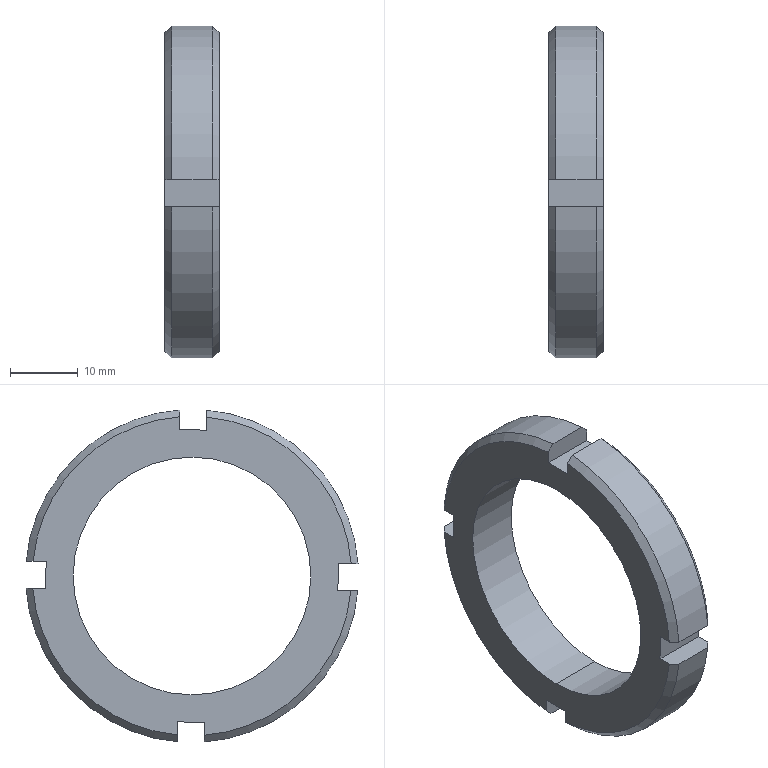Component | SolidWorks | 2-10-10WorkpieceAxisAssembly-1_2-10-5LockNut-1 | 1 solid | 28 faces | box 8 x 48.87 x 48.87 mm | volume 6873 mm3 | plane 14 | cone 8 | cylinder 6 | commonest cylinder face diameters 49 x4 35 x2
STEP:
#1=CARTESIAN_POINT('',(-19.953,-0.1704,0.689));
#2=VERTEX_POINT('',#1);
#3=CARTESIAN_POINT('',(-19.953,-0.1588,-0.689));
#4=VERTEX_POINT('',#3);
#5=CARTESIAN_POINT('',(-19.953,-0.1646,-0.));
#6=DIRECTION('',(1.,-0.,0.));
#7=DIRECTION('',(0.,0.008395,-1.));
#8=AXIS2_PLACEMENT_3D('',#5,#6,#7);
#9=CIRCLE('',#8,0.689);
#10=EDGE_CURVE('',#2,#4,#9,.T.);
#11=ORIENTED_EDGE('',*,*,#10,.F.);
#12=CARTESIAN_POINT('',(-19.638,-0.1704,0.689));
#13=VERTEX_POINT('',#12);
#14=CARTESIAN_POINT('',(-19.638,-0.1704,0.689));
#15=DIRECTION('',(1.,-0.,0.));
#16=VECTOR('',#15,39.37);
#17=LINE('',#14,#16);
#18=EDGE_CURVE('',#2,#13,#17,.T.);
#19=ORIENTED_EDGE('',*,*,#18,.T.);
#20=CARTESIAN_POINT('',(-19.638,-0.1588,-0.689));
#21=VERTEX_POINT('',#20);
#22=CARTESIAN_POINT('',(-19.638,-0.1646,-0.));
#23=DIRECTION('',(1.,-0.,0.));
#24=DIRECTION('',(0.,0.008395,-1.));
#25=AXIS2_PLACEMENT_3D('',#22,#23,#24);
#26=CIRCLE('',#25,0.689);
#27=EDGE_CURVE('',#13,#21,#26,.T.);
#28=ORIENTED_EDGE('',*,*,#27,.T.);
#29=CARTESIAN_POINT('',(-19.638,-0.1588,-0.689));
#30=DIRECTION('',(1.,-0.,0.));
#31=VECTOR('',#30,39.37);
#32=LINE('',#29,#31);
#33=EDGE_CURVE('',#4,#21,#32,.T.);
#34=ORIENTED_EDGE('',*,*,#33,.F.);
#35=EDGE_LOOP('',(#11,#19,#28,#34));
#36=FACE_OUTER_BOUND('',#35,.T.);
#37=CARTESIAN_POINT('',(-19.638,-0.1646,-0.));
#38=DIRECTION('',(1.,-0.,0.));
#39=DIRECTION('',(0.,0.008395,-1.));
#40=AXIS2_PLACEMENT_3D('',#37,#38,#39);
#41=CYLINDRICAL_SURFACE('',#40,0.689);
#42=ADVANCED_FACE('',(#36),#41,.F.);
#43=CARTESIAN_POINT('',(-19.678,-0.09394,0.962));
#44=VERTEX_POINT('',#43);
#45=CARTESIAN_POINT('',(-19.678,0.796,0.08681));
#46=VERTEX_POINT('',#45);
#47=CARTESIAN_POINT('',(-19.678,-0.1646,-0.));
#48=DIRECTION('',(-1.,0.,-0.));
#49=DIRECTION('',(0.,0.008395,-1.));
#50=AXIS2_PLACEMENT_3D('',#47,#48,#49);
#51=CIRCLE('',#50,0.9646);
#52=EDGE_CURVE('',#44,#46,#51,.T.);
#53=ORIENTED_EDGE('',*,*,#52,.T.);
#54=CARTESIAN_POINT('',(-19.914,0.796,0.08681));
#55=VERTEX_POINT('',#54);
#56=CARTESIAN_POINT('',(-19.638,0.796,0.08681));
#57=DIRECTION('',(-1.,0.,-0.));
#58=VECTOR('',#57,39.37);
#59=LINE('',#56,#58);
#60=EDGE_CURVE('',#46,#55,#59,.T.);
#61=ORIENTED_EDGE('',*,*,#60,.T.);
#62=CARTESIAN_POINT('',(-19.914,-0.09394,0.962));
#63=VERTEX_POINT('',#62);
#64=CARTESIAN_POINT('',(-19.914,-0.1646,-0.));
#65=DIRECTION('',(1.,-0.,0.));
#66=DIRECTION('',(0.,0.008395,-1.));
#67=AXIS2_PLACEMENT_3D('',#64,#65,#66);
#68=CIRCLE('',#67,0.9646);
#69=EDGE_CURVE('',#55,#63,#68,.T.);
#70=ORIENTED_EDGE('',*,*,#69,.T.);
#71=CARTESIAN_POINT('',(-19.638,-0.09394,0.962));
#72=DIRECTION('',(1.,-0.,0.));
#73=VECTOR('',#72,39.37);
#74=LINE('',#71,#73);
#75=EDGE_CURVE('',#63,#44,#74,.T.);
#76=ORIENTED_EDGE('',*,*,#75,.T.);
#77=EDGE_LOOP('',(#53,#61,#70,#76));
#78=FACE_OUTER_BOUND('',#77,.T.);
#79=CARTESIAN_POINT('',(-19.638,-0.1646,-0.));
#80=DIRECTION('',(-1.,0.,-0.));
#81=DIRECTION('',(0.,-0.008395,1.));
#82=AXIS2_PLACEMENT_3D('',#79,#80,#81);
#83=CYLINDRICAL_SURFACE('',#82,0.9646);
#84=ADVANCED_FACE('',(#78),#83,.T.);
#85=CARTESIAN_POINT('',(-19.953,0.7565,0.08648));
#86=VERTEX_POINT('',#85);
#87=CARTESIAN_POINT('',(-19.953,0.7565,0.08648));
#88=CARTESIAN_POINT('',(-19.95,0.7596,0.0865));
#89=CARTESIAN_POINT('',(-19.947,0.7626,0.08653));
#90=CARTESIAN_POINT('',(-19.944,0.7656,0.08655));
#91=CARTESIAN_POINT('',(-19.934,0.7757,0.08664));
#92=CARTESIAN_POINT('',(-19.924,0.7859,0.08672));
#93=CARTESIAN_POINT('',(-19.914,0.796,0.08681));
#94=B_SPLINE_CURVE_WITH_KNOTS('',3,(#87,#88,#89,#90,#91,#92,#93),.UNSPECIFIED.,.F.,.F.,(4,3,4),(0.005853,0.006177,0.007269),.UNSPECIFIED.);
#95=EDGE_CURVE('',#86,#55,#94,.T.);
#96=ORIENTED_EDGE('',*,*,#95,.F.);
#97=CARTESIAN_POINT('',(-19.953,-0.09361,0.9225));
#98=VERTEX_POINT('',#97);
#99=CARTESIAN_POINT('',(-19.953,-0.1646,-0.));
#100=DIRECTION('',(-1.,0.,-0.));
#101=DIRECTION('',(0.,0.008395,-1.));
#102=AXIS2_PLACEMENT_3D('',#99,#100,#101);
#103=CIRCLE('',#102,0.9252);
#104=EDGE_CURVE('',#98,#86,#103,.T.);
#105=ORIENTED_EDGE('',*,*,#104,.F.);
#106=CARTESIAN_POINT('',(-19.914,-0.09394,0.962));
#107=CARTESIAN_POINT('',(-19.919,-0.0939,0.9568));
#108=CARTESIAN_POINT('',(-19.924,-0.09385,0.9516));
#109=CARTESIAN_POINT('',(-19.929,-0.09381,0.9463));
#110=CARTESIAN_POINT('',(-19.937,-0.09374,0.9384));
#111=CARTESIAN_POINT('',(-19.945,-0.09367,0.9304));
#112=CARTESIAN_POINT('',(-19.953,-0.09361,0.9225));
#113=B_SPLINE_CURVE_WITH_KNOTS('',3,(#106,#107,#108,#109,#110,#111,#112),.UNSPECIFIED.,.F.,.F.,(4,3,4),(0.005617,0.006177,0.007033),.UNSPECIFIED.);
#114=EDGE_CURVE('',#63,#98,#113,.T.);
#115=ORIENTED_EDGE('',*,*,#114,.F.);
#116=ORIENTED_EDGE('',*,*,#69,.F.);
#117=EDGE_LOOP('',(#96,#105,#115,#116));
#118=FACE_OUTER_BOUND('',#117,.T.);
#119=CARTESIAN_POINT('',(-19.914,-0.1646,-0.));
#120=DIRECTION('',(1.,-0.,0.));
#121=DIRECTION('',(0.,0.008395,-1.));
#122=AXIS2_PLACEMENT_3D('',#119,#120,#121);
#123=CONICAL_SURFACE('',#122,0.9646,0.7854);
#124=ADVANCED_FACE('',(#118),#123,.T.);
#125=CARTESIAN_POINT('',(-19.638,0.7565,0.08648));
#126=VERTEX_POINT('',#125);
#127=CARTESIAN_POINT('',(-19.678,0.796,0.08681));
#128=CARTESIAN_POINT('',(-19.667,0.7859,0.08672));
#129=CARTESIAN_POINT('',(-19.657,0.7757,0.08664));
#130=CARTESIAN_POINT('',(-19.647,0.7656,0.08655));
#131=CARTESIAN_POINT('',(-19.644,0.7626,0.08653));
#132=CARTESIAN_POINT('',(-19.641,0.7596,0.0865));
#133=CARTESIAN_POINT('',(-19.638,0.7565,0.08648));
#134=B_SPLINE_CURVE_WITH_KNOTS('',3,(#127,#128,#129,#130,#131,#132,#133),.UNSPECIFIED.,.F.,.F.,(4,3,4),(0.005085,0.006177,0.006502),.UNSPECIFIED.);
#135=EDGE_CURVE('',#46,#126,#134,.T.);
#136=ORIENTED_EDGE('',*,*,#135,.F.);
#137=ORIENTED_EDGE('',*,*,#52,.F.);
#138=CARTESIAN_POINT('',(-19.638,-0.09361,0.9225));
#139=VERTEX_POINT('',#138);
#140=CARTESIAN_POINT('',(-19.638,-0.09361,0.9225));
#141=CARTESIAN_POINT('',(-19.646,-0.09367,0.9304));
#142=CARTESIAN_POINT('',(-19.654,-0.09374,0.9384));
#143=CARTESIAN_POINT('',(-19.662,-0.09381,0.9463));
#144=CARTESIAN_POINT('',(-19.667,-0.09385,0.9516));
#145=CARTESIAN_POINT('',(-19.672,-0.0939,0.9568));
#146=CARTESIAN_POINT('',(-19.678,-0.09394,0.962));
#147=B_SPLINE_CURVE_WITH_KNOTS('',3,(#140,#141,#142,#143,#144,#145,#146),.UNSPECIFIED.,.F.,.F.,(4,3,4),(0.005321,0.006177,0.006738),.UNSPECIFIED.);
#148=EDGE_CURVE('',#139,#44,#147,.T.);
#149=ORIENTED_EDGE('',*,*,#148,.F.);
#150=CARTESIAN_POINT('',(-19.638,-0.1646,-0.));
#151=DIRECTION('',(1.,-0.,0.));
#152=DIRECTION('',(0.,0.008395,-1.));
#153=AXIS2_PLACEMENT_3D('',#150,#151,#152);
#154=CIRCLE('',#153,0.9252);
#155=EDGE_CURVE('',#126,#139,#154,.T.);
#156=ORIENTED_EDGE('',*,*,#155,.F.);
#157=EDGE_LOOP('',(#136,#137,#149,#156));
#158=FACE_OUTER_BOUND('',#157,.T.);
#159=CARTESIAN_POINT('',(-19.638,-0.1646,-0.));
#160=DIRECTION('',(-1.,0.,-0.));
#161=DIRECTION('',(0.,-0.008395,1.));
#162=AXIS2_PLACEMENT_3D('',#159,#160,#161);
#163=CONICAL_SURFACE('',#162,0.9252,0.7854);
#164=ADVANCED_FACE('',(#158),#163,.T.);
#165=CARTESIAN_POINT('',(-19.914,-0.0778,-0.9607));
#166=VERTEX_POINT('',#165);
#167=CARTESIAN_POINT('',(-19.914,0.7974,-0.07067));
#168=VERTEX_POINT('',#167);
#169=CARTESIAN_POINT('',(-19.914,-0.1646,-0.));
#170=DIRECTION('',(1.,-0.,0.));
#171=DIRECTION('',(0.,0.008395,-1.));
#172=AXIS2_PLACEMENT_3D('',#169,#170,#171);
#173=CIRCLE('',#172,0.9646);
#174=EDGE_CURVE('',#166,#168,#173,.T.);
#175=ORIENTED_EDGE('',*,*,#174,.T.);
#176=CARTESIAN_POINT('',(-19.678,0.7974,-0.07067));
#177=VERTEX_POINT('',#176);
#178=CARTESIAN_POINT('',(-19.638,0.7974,-0.07067));
#179=DIRECTION('',(1.,-0.,0.));
#180=VECTOR('',#179,39.37);
#181=LINE('',#178,#180);
#182=EDGE_CURVE('',#168,#177,#181,.T.);
#183=ORIENTED_EDGE('',*,*,#182,.T.);
#184=CARTESIAN_POINT('',(-19.678,-0.0778,-0.9607));
#185=VERTEX_POINT('',#184);
#186=CARTESIAN_POINT('',(-19.678,-0.1646,-0.));
#187=DIRECTION('',(-1.,0.,-0.));
#188=DIRECTION('',(0.,0.008395,-1.));
#189=AXIS2_PLACEMENT_3D('',#186,#187,#188);
#190=CIRCLE('',#189,0.9646);
#191=EDGE_CURVE('',#177,#185,#190,.T.);
#192=ORIENTED_EDGE('',*,*,#191,.T.);
#193=CARTESIAN_POINT('',(-19.638,-0.0778,-0.9607));
#194=DIRECTION('',(-1.,0.,-0.));
#195=VECTOR('',#194,39.37);
#196=LINE('',#193,#195);
#197=EDGE_CURVE('',#185,#166,#196,.T.);
#198=ORIENTED_EDGE('',*,*,#197,.T.);
#199=EDGE_LOOP('',(#175,#183,#192,#198));
#200=FACE_OUTER_BOUND('',#199,.T.);
#201=CARTESIAN_POINT('',(-19.638,-0.1646,-0.));
#202=DIRECTION('',(-1.,0.,-0.));
#203=DIRECTION('',(0.,-0.008395,1.));
#204=AXIS2_PLACEMENT_3D('',#201,#202,#203);
#205=CYLINDRICAL_SURFACE('',#204,0.9646);
#206=ADVANCED_FACE('',(#200),#205,.T.);
#207=CARTESIAN_POINT('',(-19.953,0.7579,-0.071));
#208=VERTEX_POINT('',#207);
#209=CARTESIAN_POINT('',(-19.914,0.7974,-0.07067));
#210=CARTESIAN_POINT('',(-19.924,0.7872,-0.07075));
#211=CARTESIAN_POINT('',(-19.934,0.7771,-0.07084));
#212=CARTESIAN_POINT('',(-19.944,0.7669,-0.07092));
#213=CARTESIAN_POINT('',(-19.947,0.7639,-0.07095));
#214=CARTESIAN_POINT('',(-19.95,0.7609,-0.07097));
#215=CARTESIAN_POINT('',(-19.953,0.7579,-0.071));
#216=B_SPLINE_CURVE_WITH_KNOTS('',3,(#209,#210,#211,#212,#213,#214,#215),.UNSPECIFIED.,.F.,.F.,(4,3,4),(0.005085,0.006177,0.006502),.UNSPECIFIED.);
#217=EDGE_CURVE('',#168,#208,#216,.T.);
#218=ORIENTED_EDGE('',*,*,#217,.F.);
#219=ORIENTED_EDGE('',*,*,#174,.F.);
#220=CARTESIAN_POINT('',(-19.953,-0.07813,-0.9211));
#221=VERTEX_POINT('',#220);
#222=CARTESIAN_POINT('',(-19.953,-0.07813,-0.9211));
#223=CARTESIAN_POINT('',(-19.95,-0.0781,-0.9242));
#224=CARTESIAN_POINT('',(-19.947,-0.07808,-0.9272));
#225=CARTESIAN_POINT('',(-19.944,-0.07805,-0.9302));
#226=CARTESIAN_POINT('',(-19.934,-0.07797,-0.9404));
#227=CARTESIAN_POINT('',(-19.924,-0.07788,-0.9505));
#228=CARTESIAN_POINT('',(-19.914,-0.0778,-0.9607));
#229=B_SPLINE_CURVE_WITH_KNOTS('',3,(#222,#223,#224,#225,#226,#227,#228),.UNSPECIFIED.,.F.,.F.,(4,3,4),(0.005853,0.006177,0.007269),.UNSPECIFIED.);
#230=EDGE_CURVE('',#221,#166,#229,.T.);
#231=ORIENTED_EDGE('',*,*,#230,.F.);
#232=CARTESIAN_POINT('',(-19.953,-0.1646,-0.));
#233=DIRECTION('',(-1.,0.,-0.));
#234=DIRECTION('',(0.,0.008395,-1.));
#235=AXIS2_PLACEMENT_3D('',#232,#233,#234);
#236=CIRCLE('',#235,0.9252);
#237=EDGE_CURVE('',#208,#221,#236,.T.);
#238=ORIENTED_EDGE('',*,*,#237,.F.);
#239=EDGE_LOOP('',(#218,#219,#231,#238));
#240=FACE_OUTER_BOUND('',#239,.T.);
#241=CARTESIAN_POINT('',(-19.914,-0.1646,-0.));
#242=DIRECTION('',(1.,-0.,0.));
#243=DIRECTION('',(0.,0.008395,-1.));
#244=AXIS2_PLACEMENT_3D('',#241,#242,#243);
#245=CONICAL_SURFACE('',#244,0.9646,0.7854);
#246=ADVANCED_FACE('',(#240),#245,.T.);
#247=CARTESIAN_POINT('',(-19.638,0.7579,-0.071));
#248=VERTEX_POINT('',#247);
#249=CARTESIAN_POINT('',(-19.638,0.7579,-0.071));
#250=CARTESIAN_POINT('',(-19.641,0.7609,-0.07097));
#251=CARTESIAN_POINT('',(-19.644,0.7639,-0.07095));
#252=CARTESIAN_POINT('',(-19.647,0.7669,-0.07092));
#253=CARTESIAN_POINT('',(-19.657,0.7771,-0.07084));
#254=CARTESIAN_POINT('',(-19.667,0.7872,-0.07075));
#255=CARTESIAN_POINT('',(-19.678,0.7974,-0.07067));
#256=B_SPLINE_CURVE_WITH_KNOTS('',3,(#249,#250,#251,#252,#253,#254,#255),.UNSPECIFIED.,.F.,.F.,(4,3,4),(0.005853,0.006177,0.007269),.UNSPECIFIED.);
#257=EDGE_CURVE('',#248,#177,#256,.T.);
#258=ORIENTED_EDGE('',*,*,#257,.F.);
#259=CARTESIAN_POINT('',(-19.638,-0.07813,-0.9211));
#260=VERTEX_POINT('',#259);
#261=CARTESIAN_POINT('',(-19.638,-0.1646,-0.));
#262=DIRECTION('',(1.,-0.,0.));
#263=DIRECTION('',(0.,0.008395,-1.));
#264=AXIS2_PLACEMENT_3D('',#261,#262,#263);
#265=CIRCLE('',#264,0.9252);
#266=EDGE_CURVE('',#260,#248,#265,.T.);
#267=ORIENTED_EDGE('',*,*,#266,.F.);
#268=CARTESIAN_POINT('',(-19.678,-0.0778,-0.9607));
#269=CARTESIAN_POINT('',(-19.667,-0.07788,-0.9505));
#270=CARTESIAN_POINT('',(-19.657,-0.07797,-0.9404));
#271=CARTESIAN_POINT('',(-19.647,-0.07805,-0.9302));
#272=CARTESIAN_POINT('',(-19.644,-0.07808,-0.9272));
#273=CARTESIAN_POINT('',(-19.641,-0.0781,-0.9242));
#274=CARTESIAN_POINT('',(-19.638,-0.07813,-0.9211));
#275=B_SPLINE_CURVE_WITH_KNOTS('',3,(#268,#269,#270,#271,#272,#273,#274),.UNSPECIFIED.,.F.,.F.,(4,3,4),(0.005085,0.006177,0.006502),.UNSPECIFIED.);
#276=EDGE_CURVE('',#185,#260,#275,.T.);
#277=ORIENTED_EDGE('',*,*,#276,.F.);
#278=ORIENTED_EDGE('',*,*,#191,.F.);
#279=EDGE_LOOP('',(#258,#267,#277,#278));
#280=FACE_OUTER_BOUND('',#279,.T.);
#281=CARTESIAN_POINT('',(-19.638,-0.1646,-0.));
#282=DIRECTION('',(-1.,0.,-0.));
#283=DIRECTION('',(0.,-0.008395,1.));
#284=AXIS2_PLACEMENT_3D('',#281,#282,#283);
#285=CONICAL_SURFACE('',#284,0.9252,0.7854);
#286=ADVANCED_FACE('',(#280),#285,.T.);
#287=CARTESIAN_POINT('',(-19.914,-1.125,-0.08681));
#288=VERTEX_POINT('',#287);
#289=CARTESIAN_POINT('',(-19.914,-0.2353,-0.962));
#290=VERTEX_POINT('',#289);
#291=CARTESIAN_POINT('',(-19.914,-0.1646,-0.));
#292=DIRECTION('',(1.,-0.,0.));
#293=DIRECTION('',(0.,0.008395,-1.));
#294=AXIS2_PLACEMENT_3D('',#291,#292,#293);
#295=CIRCLE('',#294,0.9646);
#296=EDGE_CURVE('',#288,#290,#295,.T.);
#297=ORIENTED_EDGE('',*,*,#296,.T.);
#298=CARTESIAN_POINT('',(-19.678,-0.2353,-0.962));
#299=VERTEX_POINT('',#298);
#300=CARTESIAN_POINT('',(-19.638,-0.2353,-0.962));
#301=DIRECTION('',(1.,-0.,0.));
#302=VECTOR('',#301,39.37);
#303=LINE('',#300,#302);
#304=EDGE_CURVE('',#290,#299,#303,.T.);
#305=ORIENTED_EDGE('',*,*,#304,.T.);
#306=CARTESIAN_POINT('',(-19.678,-1.125,-0.08681));
#307=VERTEX_POINT('',#306);
#308=CARTESIAN_POINT('',(-19.678,-0.1646,-0.));
#309=DIRECTION('',(-1.,0.,-0.));
#310=DIRECTION('',(0.,0.008395,-1.));
#311=AXIS2_PLACEMENT_3D('',#308,#309,#310);
#312=CIRCLE('',#311,0.9646);
#313=EDGE_CURVE('',#299,#307,#312,.T.);
#314=ORIENTED_EDGE('',*,*,#313,.T.);
#315=CARTESIAN_POINT('',(-19.638,-1.125,-0.08681));
#316=DIRECTION('',(-1.,0.,-0.));
#317=VECTOR('',#316,39.37);
#318=LINE('',#315,#317);
#319=EDGE_CURVE('',#307,#288,#318,.T.);
#320=ORIENTED_EDGE('',*,*,#319,.T.);
#321=EDGE_LOOP('',(#297,#305,#314,#320));
#322=FACE_OUTER_BOUND('',#321,.T.);
#323=CARTESIAN_POINT('',(-19.638,-0.1646,-0.));
#324=DIRECTION('',(-1.,0.,-0.));
#325=DIRECTION('',(0.,-0.008395,1.));
#326=AXIS2_PLACEMENT_3D('',#323,#324,#325);
#327=CYLINDRICAL_SURFACE('',#326,0.9646);
#328=ADVANCED_FACE('',(#322),#327,.T.);
#329=CARTESIAN_POINT('',(-19.953,-0.2356,-0.9225));
#330=VERTEX_POINT('',#329);
#331=CARTESIAN_POINT('',(-19.914,-0.2353,-0.962));
#332=CARTESIAN_POINT('',(-19.924,-0.2354,-0.9518));
#333=CARTESIAN_POINT('',(-19.934,-0.2354,-0.9417));
#334=CARTESIAN_POINT('',(-19.944,-0.2355,-0.9315));
#335=CARTESIAN_POINT('',(-19.947,-0.2356,-0.9285));
#336=CARTESIAN_POINT('',(-19.95,-0.2356,-0.9255));
#337=CARTESIAN_POINT('',(-19.953,-0.2356,-0.9225));
#338=B_SPLINE_CURVE_WITH_KNOTS('',3,(#331,#332,#333,#334,#335,#336,#337),.UNSPECIFIED.,.F.,.F.,(4,3,4),(0.005085,0.006177,0.006502),.UNSPECIFIED.);
#339=EDGE_CURVE('',#290,#330,#338,.T.);
#340=ORIENTED_EDGE('',*,*,#339,.F.);
#341=ORIENTED_EDGE('',*,*,#296,.F.);
#342=CARTESIAN_POINT('',(-19.953,-1.086,-0.08648));
#343=VERTEX_POINT('',#342);
#344=CARTESIAN_POINT('',(-19.953,-1.086,-0.08648));
#345=CARTESIAN_POINT('',(-19.945,-1.094,-0.08654));
#346=CARTESIAN_POINT('',(-19.937,-1.102,-0.08661));
#347=CARTESIAN_POINT('',(-19.929,-1.11,-0.08668));
#348=CARTESIAN_POINT('',(-19.924,-1.115,-0.08672));
#349=CARTESIAN_POINT('',(-19.919,-1.12,-0.08676));
#350=CARTESIAN_POINT('',(-19.914,-1.125,-0.08681));
#351=B_SPLINE_CURVE_WITH_KNOTS('',3,(#344,#345,#346,#347,#348,#349,#350),.UNSPECIFIED.,.F.,.F.,(4,3,4),(0.005321,0.006177,0.006738),.UNSPECIFIED.);
#352=EDGE_CURVE('',#343,#288,#351,.T.);
#353=ORIENTED_EDGE('',*,*,#352,.F.);
#354=CARTESIAN_POINT('',(-19.953,-0.1646,-0.));
#355=DIRECTION('',(-1.,0.,-0.));
#356=DIRECTION('',(0.,0.008395,-1.));
#357=AXIS2_PLACEMENT_3D('',#354,#355,#356);
#358=CIRCLE('',#357,0.9252);
#359=EDGE_CURVE('',#330,#343,#358,.T.);
#360=ORIENTED_EDGE('',*,*,#359,.F.);
#361=EDGE_LOOP('',(#340,#341,#353,#360));
#362=FACE_OUTER_BOUND('',#361,.T.);
#363=CARTESIAN_POINT('',(-19.914,-0.1646,-0.));
#364=DIRECTION('',(1.,-0.,0.));
#365=DIRECTION('',(0.,0.008395,-1.));
#366=AXIS2_PLACEMENT_3D('',#363,#364,#365);
#367=CONICAL_SURFACE('',#366,0.9646,0.7854);
#368=ADVANCED_FACE('',(#362),#367,.T.);
#369=CARTESIAN_POINT('',(-19.638,-0.2356,-0.9225));
#370=VERTEX_POINT('',#369);
#371=CARTESIAN_POINT('',(-19.638,-0.2356,-0.9225));
#372=CARTESIAN_POINT('',(-19.641,-0.2356,-0.9255));
#373=CARTESIAN_POINT('',(-19.644,-0.2356,-0.9285));
#374=CARTESIAN_POINT('',(-19.647,-0.2355,-0.9315));
#375=CARTESIAN_POINT('',(-19.657,-0.2354,-0.9417));
#376=CARTESIAN_POINT('',(-19.667,-0.2354,-0.9518));
#377=CARTESIAN_POINT('',(-19.678,-0.2353,-0.962));
#378=B_SPLINE_CURVE_WITH_KNOTS('',3,(#371,#372,#373,#374,#375,#376,#377),.UNSPECIFIED.,.F.,.F.,(4,3,4),(0.005853,0.006177,0.007269),.UNSPECIFIED.);
#379=EDGE_CURVE('',#370,#299,#378,.T.);
#380=ORIENTED_EDGE('',*,*,#379,.F.);
#381=CARTESIAN_POINT('',(-19.638,-1.086,-0.08648));
#382=VERTEX_POINT('',#381);
#383=CARTESIAN_POINT('',(-19.638,-0.1646,-0.));
#384=DIRECTION('',(1.,-0.,0.));
#385=DIRECTION('',(0.,0.008395,-1.));
#386=AXIS2_PLACEMENT_3D('',#383,#384,#385);
#387=CIRCLE('',#386,0.9252);
#388=EDGE_CURVE('',#382,#370,#387,.T.);
#389=ORIENTED_EDGE('',*,*,#388,.F.);
#390=CARTESIAN_POINT('',(-19.678,-1.125,-0.08681));
#391=CARTESIAN_POINT('',(-19.672,-1.12,-0.08676));
#392=CARTESIAN_POINT('',(-19.667,-1.115,-0.08672));
#393=CARTESIAN_POINT('',(-19.662,-1.11,-0.08668));
#394=CARTESIAN_POINT('',(-19.654,-1.102,-0.08661));
#395=CARTESIAN_POINT('',(-19.646,-1.094,-0.08654));
#396=CARTESIAN_POINT('',(-19.638,-1.086,-0.08648));
#397=B_SPLINE_CURVE_WITH_KNOTS('',3,(#390,#391,#392,#393,#394,#395,#396),.UNSPECIFIED.,.F.,.F.,(4,3,4),(0.005617,0.006177,0.007033),.UNSPECIFIED.);
#398=EDGE_CURVE('',#307,#382,#397,.T.);
#399=ORIENTED_EDGE('',*,*,#398,.F.);
#400=ORIENTED_EDGE('',*,*,#313,.F.);
#401=EDGE_LOOP('',(#380,#389,#399,#400));
#402=FACE_OUTER_BOUND('',#401,.T.);
#403=CARTESIAN_POINT('',(-19.638,-0.1646,-0.));
#404=DIRECTION('',(-1.,0.,-0.));
#405=DIRECTION('',(0.,-0.008395,1.));
#406=AXIS2_PLACEMENT_3D('',#403,#404,#405);
#407=CONICAL_SURFACE('',#406,0.9252,0.7854);
#408=ADVANCED_FACE('',(#402),#407,.T.);
#409=CARTESIAN_POINT('',(-19.914,-0.2514,0.9607));
#410=VERTEX_POINT('',#409);
#411=CARTESIAN_POINT('',(-19.914,-1.127,0.07067));
#412=VERTEX_POINT('',#411);
#413=CARTESIAN_POINT('',(-19.914,-0.1646,-0.));
#414=DIRECTION('',(1.,-0.,0.));
#415=DIRECTION('',(0.,0.008395,-1.));
#416=AXIS2_PLACEMENT_3D('',#413,#414,#415);
#417=CIRCLE('',#416,0.9646);
#418=EDGE_CURVE('',#410,#412,#417,.T.);
#419=ORIENTED_EDGE('',*,*,#418,.T.);
#420=CARTESIAN_POINT('',(-19.678,-1.127,0.07067));
#421=VERTEX_POINT('',#420);
#422=CARTESIAN_POINT('',(-19.638,-1.127,0.07067));
#423=DIRECTION('',(1.,-0.,0.));
#424=VECTOR('',#423,39.37);
#425=LINE('',#422,#424);
#426=EDGE_CURVE('',#412,#421,#425,.T.);
#427=ORIENTED_EDGE('',*,*,#426,.T.);
#428=CARTESIAN_POINT('',(-19.678,-0.2514,0.9607));
#429=VERTEX_POINT('',#428);
#430=CARTESIAN_POINT('',(-19.678,-0.1646,-0.));
#431=DIRECTION('',(-1.,0.,-0.));
#432=DIRECTION('',(0.,0.008395,-1.));
#433=AXIS2_PLACEMENT_3D('',#430,#431,#432);
#434=CIRCLE('',#433,0.9646);
#435=EDGE_CURVE('',#421,#429,#434,.T.);
#436=ORIENTED_EDGE('',*,*,#435,.T.);
#437=CARTESIAN_POINT('',(-19.638,-0.2514,0.9607));
#438=DIRECTION('',(-1.,0.,-0.));
#439=VECTOR('',#438,39.37);
#440=LINE('',#437,#439);
#441=EDGE_CURVE('',#429,#410,#440,.T.);
#442=ORIENTED_EDGE('',*,*,#441,.T.);
#443=EDGE_LOOP('',(#419,#427,#436,#442));
#444=FACE_OUTER_BOUND('',#443,.T.);
#445=CARTESIAN_POINT('',(-19.638,-0.1646,-0.));
#446=DIRECTION('',(-1.,0.,-0.));
#447=DIRECTION('',(0.,-0.008395,1.));
#448=AXIS2_PLACEMENT_3D('',#445,#446,#447);
#449=CYLINDRICAL_SURFACE('',#448,0.9646);
#450=ADVANCED_FACE('',(#444),#449,.T.);
#451=CARTESIAN_POINT('',(-19.638,0.6812,0.08584));
#452=VERTEX_POINT('',#451);
#453=CARTESIAN_POINT('',(-19.638,1.156,0.08983));
#454=DIRECTION('',(-0.,-1.,-0.008395));
#455=VECTOR('',#454,39.37);
#456=LINE('',#453,#455);
#457=EDGE_CURVE('',#126,#452,#456,.T.);
#458=ORIENTED_EDGE('',*,*,#457,.F.);
#459=ORIENTED_EDGE('',*,*,#155,.T.);
#460=CARTESIAN_POINT('',(-19.638,-0.09297,0.8471));
#461=VERTEX_POINT('',#460);
#462=CARTESIAN_POINT('',(-19.638,-0.09696,1.322));
#463=DIRECTION('',(-0.,-0.008395,1.));
#464=VECTOR('',#463,39.37);
#465=LINE('',#462,#464);
#466=EDGE_CURVE('',#461,#139,#465,.T.);
#467=ORIENTED_EDGE('',*,*,#466,.F.);
#468=CARTESIAN_POINT('',(-19.638,-0.2504,0.8458));
#469=VERTEX_POINT('',#468);
#470=CARTESIAN_POINT('',(-19.638,-0.2504,0.8458));
#471=DIRECTION('',(0.,1.,0.008395));
#472=VECTOR('',#471,39.37);
#473=LINE('',#470,#472);
#474=EDGE_CURVE('',#469,#461,#473,.T.);
#475=ORIENTED_EDGE('',*,*,#474,.F.);
#476=CARTESIAN_POINT('',(-19.638,-0.2511,0.9211));
#477=VERTEX_POINT('',#476);
#478=CARTESIAN_POINT('',(-19.638,-0.2544,1.32));
#479=DIRECTION('',(0.,0.008395,-1.));
#480=VECTOR('',#479,39.37);
#481=LINE('',#478,#480);
#482=EDGE_CURVE('',#477,#469,#481,.T.);
#483=ORIENTED_EDGE('',*,*,#482,.F.);
#484=CARTESIAN_POINT('',(-19.638,-1.087,0.071));
#485=VERTEX_POINT('',#484);
#486=CARTESIAN_POINT('',(-19.638,-0.1646,-0.));
#487=DIRECTION('',(1.,-0.,0.));
#488=DIRECTION('',(0.,0.008395,-1.));
#489=AXIS2_PLACEMENT_3D('',#486,#487,#488);
#490=CIRCLE('',#489,0.9252);
#491=EDGE_CURVE('',#477,#485,#490,.T.);
#492=ORIENTED_EDGE('',*,*,#491,.T.);
#493=CARTESIAN_POINT('',(-19.638,-1.012,0.07163));
#494=VERTEX_POINT('',#493);
#495=CARTESIAN_POINT('',(-19.638,-1.486,0.06765));
#496=DIRECTION('',(-0.,-1.,-0.008395));
#497=VECTOR('',#496,39.37);
#498=LINE('',#495,#497);
#499=EDGE_CURVE('',#494,#485,#498,.T.);
#500=ORIENTED_EDGE('',*,*,#499,.F.);
#501=CARTESIAN_POINT('',(-19.638,-1.01,-0.08584));
#502=VERTEX_POINT('',#501);
#503=CARTESIAN_POINT('',(-19.638,-1.01,-0.08584));
#504=DIRECTION('',(-0.,-0.008395,1.));
#505=VECTOR('',#504,39.37);
#506=LINE('',#503,#505);
#507=EDGE_CURVE('',#502,#494,#506,.T.);
#508=ORIENTED_EDGE('',*,*,#507,.F.);
#509=CARTESIAN_POINT('',(-19.638,-1.485,-0.08983));
#510=DIRECTION('',(0.,1.,0.008395));
#511=VECTOR('',#510,39.37);
#512=LINE('',#509,#511);
#513=EDGE_CURVE('',#382,#502,#512,.T.);
#514=ORIENTED_EDGE('',*,*,#513,.F.);
#515=ORIENTED_EDGE('',*,*,#388,.T.);
#516=CARTESIAN_POINT('',(-19.638,-0.2362,-0.8471));
#517=VERTEX_POINT('',#516);
#518=CARTESIAN_POINT('',(-19.638,-0.2323,-1.322));
#519=DIRECTION('',(0.,0.008395,-1.));
#520=VECTOR('',#519,39.37);
#521=LINE('',#518,#520);
#522=EDGE_CURVE('',#517,#370,#521,.T.);
#523=ORIENTED_EDGE('',*,*,#522,.F.);
#524=CARTESIAN_POINT('',(-19.638,-0.07876,-0.8458));
#525=VERTEX_POINT('',#524);
#526=CARTESIAN_POINT('',(-19.638,-0.07876,-0.8458));
#527=DIRECTION('',(-0.,-1.,-0.008395));
#528=VECTOR('',#527,39.37);
#529=LINE('',#526,#528);
#530=EDGE_CURVE('',#525,#517,#529,.T.);
#531=ORIENTED_EDGE('',*,*,#530,.F.);
#532=CARTESIAN_POINT('',(-19.638,-0.07478,-1.32));
#533=DIRECTION('',(-0.,-0.008395,1.));
#534=VECTOR('',#533,39.37);
#535=LINE('',#532,#534);
#536=EDGE_CURVE('',#260,#525,#535,.T.);
#537=ORIENTED_EDGE('',*,*,#536,.F.);
#538=ORIENTED_EDGE('',*,*,#266,.T.);
#539=CARTESIAN_POINT('',(-19.638,0.6825,-0.07163));
#540=VERTEX_POINT('',#539);
#541=CARTESIAN_POINT('',(-19.638,1.157,-0.06765));
#542=DIRECTION('',(0.,1.,0.008395));
#543=VECTOR('',#542,39.37);
#544=LINE('',#541,#543);
#545=EDGE_CURVE('',#540,#248,#544,.T.);
#546=ORIENTED_EDGE('',*,*,#545,.F.);
#547=CARTESIAN_POINT('',(-19.638,0.6812,0.08584));
#548=DIRECTION('',(0.,0.008395,-1.));
#549=VECTOR('',#548,39.37);
#550=LINE('',#547,#549);
#551=EDGE_CURVE('',#452,#540,#550,.T.);
#552=ORIENTED_EDGE('',*,*,#551,.F.);
#553=EDGE_LOOP('',(#458,#459,#467,#475,#483,#492,#500,#508,#514,#515,#523,#531,#537,#538,#546,#552));
#554=FACE_OUTER_BOUND('',#553,.T.);
#555=CARTESIAN_POINT('',(-19.638,-0.1646,-0.));
#556=DIRECTION('',(1.,-0.,0.));
#557=DIRECTION('',(0.,0.008395,-1.));
#558=AXIS2_PLACEMENT_3D('',#555,#556,#557);
#559=CIRCLE('',#558,0.689);
#560=EDGE_CURVE('',#21,#13,#559,.T.);
#561=ORIENTED_EDGE('',*,*,#560,.F.);
#562=ORIENTED_EDGE('',*,*,#27,.F.);
#563=EDGE_LOOP('',(#561,#562));
#564=FACE_BOUND('',#563,.T.);
#565=CARTESIAN_POINT('',(-19.638,-0.1646,-0.));
#566=DIRECTION('',(1.,-0.,0.));
#567=DIRECTION('',(0.,0.008395,-1.));
#568=AXIS2_PLACEMENT_3D('',#565,#566,#567);
#569=PLANE('',#568);
#570=ADVANCED_FACE('',(#554,#564),#569,.T.);
#571=ORIENTED_EDGE('',*,*,#104,.T.);
#572=CARTESIAN_POINT('',(-19.953,0.6812,0.08584));
#573=VERTEX_POINT('',#572);
#574=CARTESIAN_POINT('',(-19.953,-0.1653,0.07874));
#575=DIRECTION('',(-0.,-1.,-0.008395));
#576=VECTOR('',#575,39.37);
#577=LINE('',#574,#576);
#578=EDGE_CURVE('',#86,#573,#577,.T.);
#579=ORIENTED_EDGE('',*,*,#578,.T.);
#580=CARTESIAN_POINT('',(-19.953,0.6825,-0.07163));
#581=VERTEX_POINT('',#580);
#582=CARTESIAN_POINT('',(-19.953,0.6818,0.007106));
#583=DIRECTION('',(0.,0.008395,-1.));
#584=VECTOR('',#583,39.37);
#585=LINE('',#582,#584);
#586=EDGE_CURVE('',#573,#581,#585,.T.);
#587=ORIENTED_EDGE('',*,*,#586,.T.);
#588=CARTESIAN_POINT('',(-19.953,-0.1639,-0.07874));
#589=DIRECTION('',(0.,1.,0.008395));
#590=VECTOR('',#589,39.37);
#591=LINE('',#588,#590);
#592=EDGE_CURVE('',#581,#208,#591,.T.);
#593=ORIENTED_EDGE('',*,*,#592,.T.);
#594=ORIENTED_EDGE('',*,*,#237,.T.);
#595=CARTESIAN_POINT('',(-19.953,-0.07876,-0.8458));
#596=VERTEX_POINT('',#595);
#597=CARTESIAN_POINT('',(-19.953,-0.08587,0.000661));
#598=DIRECTION('',(-0.,-0.008395,1.));
#599=VECTOR('',#598,39.37);
#600=LINE('',#597,#599);
#601=EDGE_CURVE('',#221,#596,#600,.T.);
#602=ORIENTED_EDGE('',*,*,#601,.T.);
#603=CARTESIAN_POINT('',(-19.953,-0.2362,-0.8471));
#604=VERTEX_POINT('',#603);
#605=CARTESIAN_POINT('',(-19.953,-0.1575,-0.8464));
#606=DIRECTION('',(-0.,-1.,-0.008395));
#607=VECTOR('',#606,39.37);
#608=LINE('',#605,#607);
#609=EDGE_CURVE('',#596,#604,#608,.T.);
#610=ORIENTED_EDGE('',*,*,#609,.T.);
#611=CARTESIAN_POINT('',(-19.953,-0.2433,-0.000661));
#612=DIRECTION('',(0.,0.008395,-1.));
#613=VECTOR('',#612,39.37);
#614=LINE('',#611,#613);
#615=EDGE_CURVE('',#604,#330,#614,.T.);
#616=ORIENTED_EDGE('',*,*,#615,.T.);
#617=ORIENTED_EDGE('',*,*,#359,.T.);
#618=CARTESIAN_POINT('',(-19.953,-1.01,-0.08584));
#619=VERTEX_POINT('',#618);
#620=CARTESIAN_POINT('',(-19.953,-0.1639,-0.07874));
#621=DIRECTION('',(0.,1.,0.008395));
#622=VECTOR('',#621,39.37);
#623=LINE('',#620,#622);
#624=EDGE_CURVE('',#343,#619,#623,.T.);
#625=ORIENTED_EDGE('',*,*,#624,.T.);
#626=CARTESIAN_POINT('',(-19.953,-1.012,0.07163));
#627=VERTEX_POINT('',#626);
#628=CARTESIAN_POINT('',(-19.953,-1.011,-0.007106));
#629=DIRECTION('',(-0.,-0.008395,1.));
#630=VECTOR('',#629,39.37);
#631=LINE('',#628,#630);
#632=EDGE_CURVE('',#619,#627,#631,.T.);
#633=ORIENTED_EDGE('',*,*,#632,.T.);
#634=CARTESIAN_POINT('',(-19.953,-1.087,0.071));
#635=VERTEX_POINT('',#634);
#636=CARTESIAN_POINT('',(-19.953,-0.1653,0.07874));
#637=DIRECTION('',(-0.,-1.,-0.008395));
#638=VECTOR('',#637,39.37);
#639=LINE('',#636,#638);
#640=EDGE_CURVE('',#627,#635,#639,.T.);
#641=ORIENTED_EDGE('',*,*,#640,.T.);
#642=CARTESIAN_POINT('',(-19.953,-0.2511,0.9211));
#643=VERTEX_POINT('',#642);
#644=CARTESIAN_POINT('',(-19.953,-0.1646,-0.));
#645=DIRECTION('',(-1.,0.,-0.));
#646=DIRECTION('',(0.,0.008395,-1.));
#647=AXIS2_PLACEMENT_3D('',#644,#645,#646);
#648=CIRCLE('',#647,0.9252);
#649=EDGE_CURVE('',#635,#643,#648,.T.);
#650=ORIENTED_EDGE('',*,*,#649,.T.);
#651=CARTESIAN_POINT('',(-19.953,-0.2504,0.8458));
#652=VERTEX_POINT('',#651);
#653=CARTESIAN_POINT('',(-19.953,-0.2433,-0.000661));
#654=DIRECTION('',(0.,0.008395,-1.));
#655=VECTOR('',#654,39.37);
#656=LINE('',#653,#655);
#657=EDGE_CURVE('',#643,#652,#656,.T.);
#658=ORIENTED_EDGE('',*,*,#657,.T.);
#659=CARTESIAN_POINT('',(-19.953,-0.09297,0.8471));
#660=VERTEX_POINT('',#659);
#661=CARTESIAN_POINT('',(-19.953,-0.1717,0.8464));
#662=DIRECTION('',(0.,1.,0.008395));
#663=VECTOR('',#662,39.37);
#664=LINE('',#661,#663);
#665=EDGE_CURVE('',#652,#660,#664,.T.);
#666=ORIENTED_EDGE('',*,*,#665,.T.);
#667=CARTESIAN_POINT('',(-19.953,-0.08587,0.000661));
#668=DIRECTION('',(-0.,-0.008395,1.));
#669=VECTOR('',#668,39.37);
#670=LINE('',#667,#669);
#671=EDGE_CURVE('',#660,#98,#670,.T.);
#672=ORIENTED_EDGE('',*,*,#671,.T.);
#673=EDGE_LOOP('',(#571,#579,#587,#593,#594,#602,#610,#616,#617,#625,#633,#641,#650,#658,#666,#672));
#674=FACE_OUTER_BOUND('',#673,.T.);
#675=CARTESIAN_POINT('',(-19.953,-0.1646,-0.));
#676=DIRECTION('',(1.,-0.,0.));
#677=DIRECTION('',(0.,0.008395,-1.));
#678=AXIS2_PLACEMENT_3D('',#675,#676,#677);
#679=CIRCLE('',#678,0.689);
#680=EDGE_CURVE('',#4,#2,#679,.T.);
#681=ORIENTED_EDGE('',*,*,#680,.T.);
#682=ORIENTED_EDGE('',*,*,#10,.T.);
#683=EDGE_LOOP('',(#681,#682));
#684=FACE_BOUND('',#683,.T.);
#685=CARTESIAN_POINT('',(-19.953,-0.1646,-0.));
#686=DIRECTION('',(1.,-0.,0.));
#687=DIRECTION('',(0.,0.008395,-1.));
#688=AXIS2_PLACEMENT_3D('',#685,#686,#687);
#689=PLANE('',#688);
#690=ADVANCED_FACE('',(#674,#684),#689,.F.);
#691=CARTESIAN_POINT('',(-19.914,-1.127,0.07067));
#692=CARTESIAN_POINT('',(-19.919,-1.121,0.07071));
#693=CARTESIAN_POINT('',(-19.924,-1.116,0.07075));
#694=CARTESIAN_POINT('',(-19.929,-1.111,0.0708));
#695=CARTESIAN_POINT('',(-19.937,-1.103,0.07087));
#696=CARTESIAN_POINT('',(-19.945,-1.095,0.07093));
#697=CARTESIAN_POINT('',(-19.953,-1.087,0.071));
#698=B_SPLINE_CURVE_WITH_KNOTS('',3,(#691,#692,#693,#694,#695,#696,#697),.UNSPECIFIED.,.F.,.F.,(4,3,4),(0.005617,0.006177,0.007033),.UNSPECIFIED.);
#699=EDGE_CURVE('',#412,#635,#698,.T.);
#700=ORIENTED_EDGE('',*,*,#699,.F.);
#701=ORIENTED_EDGE('',*,*,#418,.F.);
#702=CARTESIAN_POINT('',(-19.953,-0.2511,0.9211));
#703=CARTESIAN_POINT('',(-19.945,-0.2511,0.9291));
#704=CARTESIAN_POINT('',(-19.937,-0.2512,0.9371));
#705=CARTESIAN_POINT('',(-19.929,-0.2513,0.945));
#706=CARTESIAN_POINT('',(-19.924,-0.2513,0.9502));
#707=CARTESIAN_POINT('',(-19.919,-0.2514,0.9554));
#708=CARTESIAN_POINT('',(-19.914,-0.2514,0.9607));
#709=B_SPLINE_CURVE_WITH_KNOTS('',3,(#702,#703,#704,#705,#706,#707,#708),.UNSPECIFIED.,.F.,.F.,(4,3,4),(0.005321,0.006177,0.006738),.UNSPECIFIED.);
#710=EDGE_CURVE('',#643,#410,#709,.T.);
#711=ORIENTED_EDGE('',*,*,#710,.F.);
#712=ORIENTED_EDGE('',*,*,#649,.F.);
#713=EDGE_LOOP('',(#700,#701,#711,#712));
#714=FACE_OUTER_BOUND('',#713,.T.);
#715=CARTESIAN_POINT('',(-19.914,-0.1646,-0.));
#716=DIRECTION('',(1.,-0.,0.));
#717=DIRECTION('',(0.,0.008395,-1.));
#718=AXIS2_PLACEMENT_3D('',#715,#716,#717);
#719=CONICAL_SURFACE('',#718,0.9646,0.7854);
#720=ADVANCED_FACE('',(#714),#719,.T.);
#721=CARTESIAN_POINT('',(-19.638,-1.087,0.071));
#722=CARTESIAN_POINT('',(-19.646,-1.095,0.07093));
#723=CARTESIAN_POINT('',(-19.654,-1.103,0.07087));
#724=CARTESIAN_POINT('',(-19.662,-1.111,0.0708));
#725=CARTESIAN_POINT('',(-19.667,-1.116,0.07075));
#726=CARTESIAN_POINT('',(-19.672,-1.121,0.07071));
#727=CARTESIAN_POINT('',(-19.678,-1.127,0.07067));
#728=B_SPLINE_CURVE_WITH_KNOTS('',3,(#721,#722,#723,#724,#725,#726,#727),.UNSPECIFIED.,.F.,.F.,(4,3,4),(0.005321,0.006177,0.006738),.UNSPECIFIED.);
#729=EDGE_CURVE('',#485,#421,#728,.T.);
#730=ORIENTED_EDGE('',*,*,#729,.F.);
#731=ORIENTED_EDGE('',*,*,#491,.F.);
#732=CARTESIAN_POINT('',(-19.678,-0.2514,0.9607));
#733=CARTESIAN_POINT('',(-19.672,-0.2514,0.9554));
#734=CARTESIAN_POINT('',(-19.667,-0.2513,0.9502));
#735=CARTESIAN_POINT('',(-19.662,-0.2513,0.945));
#736=CARTESIAN_POINT('',(-19.654,-0.2512,0.9371));
#737=CARTESIAN_POINT('',(-19.646,-0.2511,0.9291));
#738=CARTESIAN_POINT('',(-19.638,-0.2511,0.9211));
#739=B_SPLINE_CURVE_WITH_KNOTS('',3,(#732,#733,#734,#735,#736,#737,#738),.UNSPECIFIED.,.F.,.F.,(4,3,4),(0.005617,0.006177,0.007033),.UNSPECIFIED.);
#740=EDGE_CURVE('',#429,#477,#739,.T.);
#741=ORIENTED_EDGE('',*,*,#740,.F.);
#742=ORIENTED_EDGE('',*,*,#435,.F.);
#743=EDGE_LOOP('',(#730,#731,#741,#742));
#744=FACE_OUTER_BOUND('',#743,.T.);
#745=CARTESIAN_POINT('',(-19.638,-0.1646,-0.));
#746=DIRECTION('',(-1.,0.,-0.));
#747=DIRECTION('',(0.,-0.008395,1.));
#748=AXIS2_PLACEMENT_3D('',#745,#746,#747);
#749=CONICAL_SURFACE('',#748,0.9252,0.7854);
#750=ADVANCED_FACE('',(#744),#749,.T.);
#751=ORIENTED_EDGE('',*,*,#18,.F.);
#752=ORIENTED_EDGE('',*,*,#680,.F.);
#753=ORIENTED_EDGE('',*,*,#33,.T.);
#754=ORIENTED_EDGE('',*,*,#560,.T.);
#755=EDGE_LOOP('',(#751,#752,#753,#754));
#756=FACE_OUTER_BOUND('',#755,.T.);
#757=CARTESIAN_POINT('',(-19.638,-0.1646,-0.));
#758=DIRECTION('',(1.,-0.,0.));
#759=DIRECTION('',(0.,0.008395,-1.));
#760=AXIS2_PLACEMENT_3D('',#757,#758,#759);
#761=CYLINDRICAL_SURFACE('',#760,0.689);
#762=ADVANCED_FACE('',(#756),#761,.F.);
#763=CARTESIAN_POINT('',(-20.662,-0.2504,0.8458));
#764=DIRECTION('',(1.,-0.,0.));
#765=VECTOR('',#764,39.37);
#766=LINE('',#763,#765);
#767=EDGE_CURVE('',#652,#469,#766,.T.);
#768=ORIENTED_EDGE('',*,*,#767,.T.);
#769=ORIENTED_EDGE('',*,*,#474,.T.);
#770=CARTESIAN_POINT('',(-20.662,-0.09297,0.8471));
#771=DIRECTION('',(1.,-0.,0.));
#772=VECTOR('',#771,39.37);
#773=LINE('',#770,#772);
#774=EDGE_CURVE('',#660,#461,#773,.T.);
#775=ORIENTED_EDGE('',*,*,#774,.F.);
#776=ORIENTED_EDGE('',*,*,#665,.F.);
#777=EDGE_LOOP('',(#768,#769,#775,#776));
#778=FACE_OUTER_BOUND('',#777,.T.);
#779=CARTESIAN_POINT('',(-20.662,-0.2504,0.8458));
#780=DIRECTION('',(0.,0.008395,-1.));
#781=DIRECTION('',(0.,1.,0.008395));
#782=AXIS2_PLACEMENT_3D('',#779,#780,#781);
#783=PLANE('',#782);
#784=ADVANCED_FACE('',(#778),#783,.F.);
#785=ORIENTED_EDGE('',*,*,#710,.T.);
#786=ORIENTED_EDGE('',*,*,#441,.F.);
#787=ORIENTED_EDGE('',*,*,#740,.T.);
#788=ORIENTED_EDGE('',*,*,#482,.T.);
#789=ORIENTED_EDGE('',*,*,#767,.F.);
#790=ORIENTED_EDGE('',*,*,#657,.F.);
#791=EDGE_LOOP('',(#785,#786,#787,#788,#789,#790));
#792=FACE_OUTER_BOUND('',#791,.T.);
#793=CARTESIAN_POINT('',(-20.662,-0.2544,1.32));
#794=DIRECTION('',(-0.,-1.,-0.008395));
#795=DIRECTION('',(0.,0.008395,-1.));
#796=AXIS2_PLACEMENT_3D('',#793,#794,#795);
#797=PLANE('',#796);
#798=ADVANCED_FACE('',(#792),#797,.F.);
#799=ORIENTED_EDGE('',*,*,#774,.T.);
#800=ORIENTED_EDGE('',*,*,#466,.T.);
#801=ORIENTED_EDGE('',*,*,#148,.T.);
#802=ORIENTED_EDGE('',*,*,#75,.F.);
#803=ORIENTED_EDGE('',*,*,#114,.T.);
#804=ORIENTED_EDGE('',*,*,#671,.F.);
#805=EDGE_LOOP('',(#799,#800,#801,#802,#803,#804));
#806=FACE_OUTER_BOUND('',#805,.T.);
#807=CARTESIAN_POINT('',(-20.662,-0.09696,1.322));
#808=DIRECTION('',(0.,1.,0.008395));
#809=DIRECTION('',(-0.,-0.008395,1.));
#810=AXIS2_PLACEMENT_3D('',#807,#808,#809);
#811=PLANE('',#810);
#812=ADVANCED_FACE('',(#806),#811,.F.);
#813=CARTESIAN_POINT('',(-20.662,-1.01,-0.08584));
#814=DIRECTION('',(1.,-0.,0.));
#815=VECTOR('',#814,39.37);
#816=LINE('',#813,#815);
#817=EDGE_CURVE('',#619,#502,#816,.T.);
#818=ORIENTED_EDGE('',*,*,#817,.T.);
#819=ORIENTED_EDGE('',*,*,#507,.T.);
#820=CARTESIAN_POINT('',(-20.662,-1.012,0.07163));
#821=DIRECTION('',(1.,-0.,0.));
#822=VECTOR('',#821,39.37);
#823=LINE('',#820,#822);
#824=EDGE_CURVE('',#627,#494,#823,.T.);
#825=ORIENTED_EDGE('',*,*,#824,.F.);
#826=ORIENTED_EDGE('',*,*,#632,.F.);
#827=EDGE_LOOP('',(#818,#819,#825,#826));
#828=FACE_OUTER_BOUND('',#827,.T.);
#829=CARTESIAN_POINT('',(-20.662,-1.01,-0.08584));
#830=DIRECTION('',(0.,1.,0.008395));
#831=DIRECTION('',(-0.,-0.008395,1.));
#832=AXIS2_PLACEMENT_3D('',#829,#830,#831);
#833=PLANE('',#832);
#834=ADVANCED_FACE('',(#828),#833,.F.);
#835=ORIENTED_EDGE('',*,*,#352,.T.);
#836=ORIENTED_EDGE('',*,*,#319,.F.);
#837=ORIENTED_EDGE('',*,*,#398,.T.);
#838=ORIENTED_EDGE('',*,*,#513,.T.);
#839=ORIENTED_EDGE('',*,*,#817,.F.);
#840=ORIENTED_EDGE('',*,*,#624,.F.);
#841=EDGE_LOOP('',(#835,#836,#837,#838,#839,#840));
#842=FACE_OUTER_BOUND('',#841,.T.);
#843=CARTESIAN_POINT('',(-20.662,-1.485,-0.08983));
#844=DIRECTION('',(0.,0.008395,-1.));
#845=DIRECTION('',(0.,1.,0.008395));
#846=AXIS2_PLACEMENT_3D('',#843,#844,#845);
#847=PLANE('',#846);
#848=ADVANCED_FACE('',(#842),#847,.F.);
#849=ORIENTED_EDGE('',*,*,#824,.T.);
#850=ORIENTED_EDGE('',*,*,#499,.T.);
#851=ORIENTED_EDGE('',*,*,#729,.T.);
#852=ORIENTED_EDGE('',*,*,#426,.F.);
#853=ORIENTED_EDGE('',*,*,#699,.T.);
#854=ORIENTED_EDGE('',*,*,#640,.F.);
#855=EDGE_LOOP('',(#849,#850,#851,#852,#853,#854));
#856=FACE_OUTER_BOUND('',#855,.T.);
#857=CARTESIAN_POINT('',(-20.662,-1.486,0.06765));
#858=DIRECTION('',(-0.,-0.008395,1.));
#859=DIRECTION('',(-0.,-1.,-0.008395));
#860=AXIS2_PLACEMENT_3D('',#857,#858,#859);
#861=PLANE('',#860);
#862=ADVANCED_FACE('',(#856),#861,.F.);
#863=CARTESIAN_POINT('',(-20.662,-0.07876,-0.8458));
#864=DIRECTION('',(1.,-0.,0.));
#865=VECTOR('',#864,39.37);
#866=LINE('',#863,#865);
#867=EDGE_CURVE('',#596,#525,#866,.T.);
#868=ORIENTED_EDGE('',*,*,#867,.T.);
#869=ORIENTED_EDGE('',*,*,#530,.T.);
#870=CARTESIAN_POINT('',(-20.662,-0.2362,-0.8471));
#871=DIRECTION('',(1.,-0.,0.));
#872=VECTOR('',#871,39.37);
#873=LINE('',#870,#872);
#874=EDGE_CURVE('',#604,#517,#873,.T.);
#875=ORIENTED_EDGE('',*,*,#874,.F.);
#876=ORIENTED_EDGE('',*,*,#609,.F.);
#877=EDGE_LOOP('',(#868,#869,#875,#876));
#878=FACE_OUTER_BOUND('',#877,.T.);
#879=CARTESIAN_POINT('',(-20.662,-0.07876,-0.8458));
#880=DIRECTION('',(-0.,-0.008395,1.));
#881=DIRECTION('',(-0.,-1.,-0.008395));
#882=AXIS2_PLACEMENT_3D('',#879,#880,#881);
#883=PLANE('',#882);
#884=ADVANCED_FACE('',(#878),#883,.F.);
#885=ORIENTED_EDGE('',*,*,#276,.T.);
#886=ORIENTED_EDGE('',*,*,#536,.T.);
#887=ORIENTED_EDGE('',*,*,#867,.F.);
#888=ORIENTED_EDGE('',*,*,#601,.F.);
#889=ORIENTED_EDGE('',*,*,#230,.T.);
#890=ORIENTED_EDGE('',*,*,#197,.F.);
#891=EDGE_LOOP('',(#885,#886,#887,#888,#889,#890));
#892=FACE_OUTER_BOUND('',#891,.T.);
#893=CARTESIAN_POINT('',(-20.662,-0.07478,-1.32));
#894=DIRECTION('',(0.,1.,0.008395));
#895=DIRECTION('',(-0.,-0.008395,1.));
#896=AXIS2_PLACEMENT_3D('',#893,#894,#895);
#897=PLANE('',#896);
#898=ADVANCED_FACE('',(#892),#897,.F.);
#899=ORIENTED_EDGE('',*,*,#379,.T.);
#900=ORIENTED_EDGE('',*,*,#304,.F.);
#901=ORIENTED_EDGE('',*,*,#339,.T.);
#902=ORIENTED_EDGE('',*,*,#615,.F.);
#903=ORIENTED_EDGE('',*,*,#874,.T.);
#904=ORIENTED_EDGE('',*,*,#522,.T.);
#905=EDGE_LOOP('',(#899,#900,#901,#902,#903,#904));
#906=FACE_OUTER_BOUND('',#905,.T.);
#907=CARTESIAN_POINT('',(-20.662,-0.2323,-1.322));
#908=DIRECTION('',(-0.,-1.,-0.008395));
#909=DIRECTION('',(0.,0.008395,-1.));
#910=AXIS2_PLACEMENT_3D('',#907,#908,#909);
#911=PLANE('',#910);
#912=ADVANCED_FACE('',(#906),#911,.F.);
#913=CARTESIAN_POINT('',(-20.662,0.6812,0.08584));
#914=DIRECTION('',(1.,-0.,0.));
#915=VECTOR('',#914,39.37);
#916=LINE('',#913,#915);
#917=EDGE_CURVE('',#573,#452,#916,.T.);
#918=ORIENTED_EDGE('',*,*,#917,.T.);
#919=ORIENTED_EDGE('',*,*,#551,.T.);
#920=CARTESIAN_POINT('',(-20.662,0.6825,-0.07163));
#921=DIRECTION('',(1.,-0.,0.));
#922=VECTOR('',#921,39.37);
#923=LINE('',#920,#922);
#924=EDGE_CURVE('',#581,#540,#923,.T.);
#925=ORIENTED_EDGE('',*,*,#924,.F.);
#926=ORIENTED_EDGE('',*,*,#586,.F.);
#927=EDGE_LOOP('',(#918,#919,#925,#926));
#928=FACE_OUTER_BOUND('',#927,.T.);
#929=CARTESIAN_POINT('',(-20.662,0.6812,0.08584));
#930=DIRECTION('',(-0.,-1.,-0.008395));
#931=DIRECTION('',(0.,0.008395,-1.));
#932=AXIS2_PLACEMENT_3D('',#929,#930,#931);
#933=PLANE('',#932);
#934=ADVANCED_FACE('',(#928),#933,.F.);
#935=ORIENTED_EDGE('',*,*,#135,.T.);
#936=ORIENTED_EDGE('',*,*,#457,.T.);
#937=ORIENTED_EDGE('',*,*,#917,.F.);
#938=ORIENTED_EDGE('',*,*,#578,.F.);
#939=ORIENTED_EDGE('',*,*,#95,.T.);
#940=ORIENTED_EDGE('',*,*,#60,.F.);
#941=EDGE_LOOP('',(#935,#936,#937,#938,#939,#940));
#942=FACE_OUTER_BOUND('',#941,.T.);
#943=CARTESIAN_POINT('',(-20.662,1.156,0.08983));
#944=DIRECTION('',(-0.,-0.008395,1.));
#945=DIRECTION('',(-0.,-1.,-0.008395));
#946=AXIS2_PLACEMENT_3D('',#943,#944,#945);
#947=PLANE('',#946);
#948=ADVANCED_FACE('',(#942),#947,.F.);
#949=ORIENTED_EDGE('',*,*,#257,.T.);
#950=ORIENTED_EDGE('',*,*,#182,.F.);
#951=ORIENTED_EDGE('',*,*,#217,.T.);
#952=ORIENTED_EDGE('',*,*,#592,.F.);
#953=ORIENTED_EDGE('',*,*,#924,.T.);
#954=ORIENTED_EDGE('',*,*,#545,.T.);
#955=EDGE_LOOP('',(#949,#950,#951,#952,#953,#954));
#956=FACE_OUTER_BOUND('',#955,.T.);
#957=CARTESIAN_POINT('',(-20.662,1.157,-0.06765));
#958=DIRECTION('',(0.,0.008395,-1.));
#959=DIRECTION('',(0.,1.,0.008395));
#960=AXIS2_PLACEMENT_3D('',#957,#958,#959);
#961=PLANE('',#960);
#962=ADVANCED_FACE('',(#956),#961,.F.);
#963=CLOSED_SHELL('',(#42,#84,#124,#164,#206,#246,#286,#328,#368,#408,#450,#570,#690,#720,#750,#762,#784,#798,#812,#834,#848,#862,#884,#898,#912,#934,#948,#962));
#964=MANIFOLD_SOLID_BREP('',#963);
#965=CARTESIAN_POINT('',(0.,0.,0.));
#966=DIRECTION('',(0.,0.,1.));
#967=DIRECTION('',(1.,0.,0.));
#968=AXIS2_PLACEMENT_3D('',#965,#966,#967);
#969=(LENGTH_UNIT()NAMED_UNIT(*)SI_UNIT($,.METRE.));
#970=LENGTH_MEASURE_WITH_UNIT(LENGTH_MEASURE(0.0254),#969);
#971=DIMENSIONAL_EXPONENTS(1.,0.,0.,0.,0.,0.,0.);
#972=(CONVERSION_BASED_UNIT('',#970)LENGTH_UNIT()NAMED_UNIT(#971));
#973=UNCERTAINTY_MEASURE_WITH_UNIT(LENGTH_MEASURE(0.00001),#972,'','');
#974=(NAMED_UNIT(*)PLANE_ANGLE_UNIT()SI_UNIT($,.RADIAN.));
#975=(NAMED_UNIT(*)SI_UNIT($,.STERADIAN.)SOLID_ANGLE_UNIT());
#976=(GEOMETRIC_REPRESENTATION_CONTEXT(3)GLOBAL_UNCERTAINTY_ASSIGNED_CONTEXT((#973))GLOBAL_UNIT_ASSIGNED_CONTEXT((#972,#974,#975))REPRESENTATION_CONTEXT('',''));
#977=ADVANCED_BREP_SHAPE_REPRESENTATION('',(#964,#968),#976);
#978=COLOUR_RGB('',0.7922,0.8196,0.9333);
#979=FILL_AREA_STYLE_COLOUR('',#978);
#980=FILL_AREA_STYLE('',(#979));
#981=SURFACE_STYLE_FILL_AREA(#980);
#982=SURFACE_SIDE_STYLE('',(#981));
#983=SURFACE_STYLE_USAGE(.BOTH.,#982);
#984=PRESENTATION_STYLE_ASSIGNMENT((#983));
#985=STYLED_ITEM('',(#984),#964);
#986=PRESENTATION_LAYER_ASSIGNMENT('','',(#985));
#987=(LENGTH_UNIT()NAMED_UNIT(*)SI_UNIT($,.METRE.));
#988=LENGTH_MEASURE_WITH_UNIT(LENGTH_MEASURE(0.0254),#987);
#989=DIMENSIONAL_EXPONENTS(1.,0.,0.,0.,0.,0.,0.);
#990=(CONVERSION_BASED_UNIT('',#988)LENGTH_UNIT()NAMED_UNIT(#989));
#991=UNCERTAINTY_MEASURE_WITH_UNIT(LENGTH_MEASURE(0.00001),#990,'','');
#992=(NAMED_UNIT(*)PLANE_ANGLE_UNIT()SI_UNIT($,.RADIAN.));
#993=(NAMED_UNIT(*)SI_UNIT($,.STERADIAN.)SOLID_ANGLE_UNIT());
#994=(GEOMETRIC_REPRESENTATION_CONTEXT(3)GLOBAL_UNCERTAINTY_ASSIGNED_CONTEXT((#991))GLOBAL_UNIT_ASSIGNED_CONTEXT((#990,#992,#993))REPRESENTATION_CONTEXT('',''));
#995=MECHANICAL_DESIGN_GEOMETRIC_PRESENTATION_REPRESENTATION('',(#985),#994);